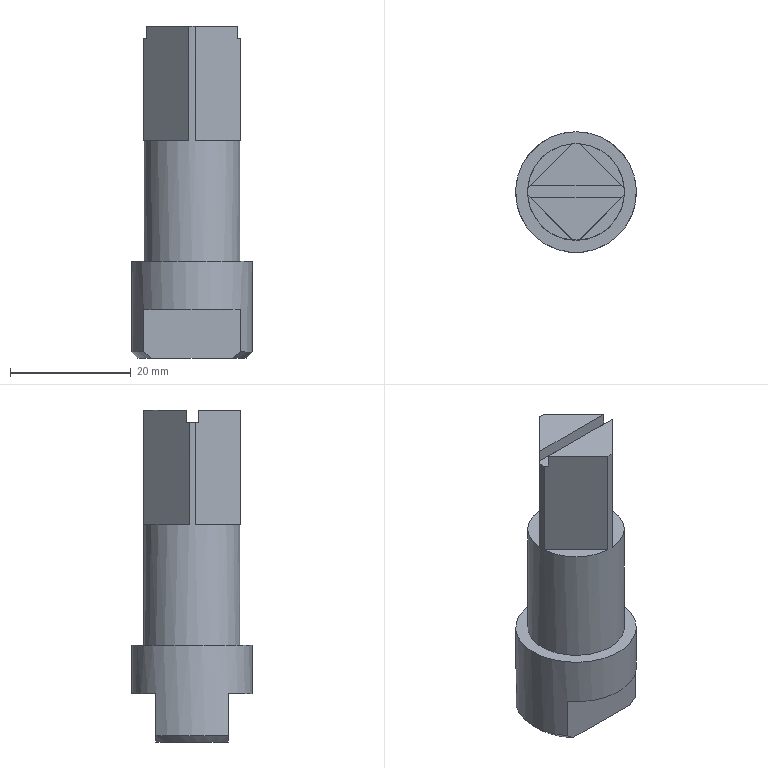Component | NX | VALVESTEM | 1 solid | 23 faces | volume 10974 mm3 | plane 19 | cylinder 2 | cone 2 | commonest cylinder face diameters 16 x1 20 x1